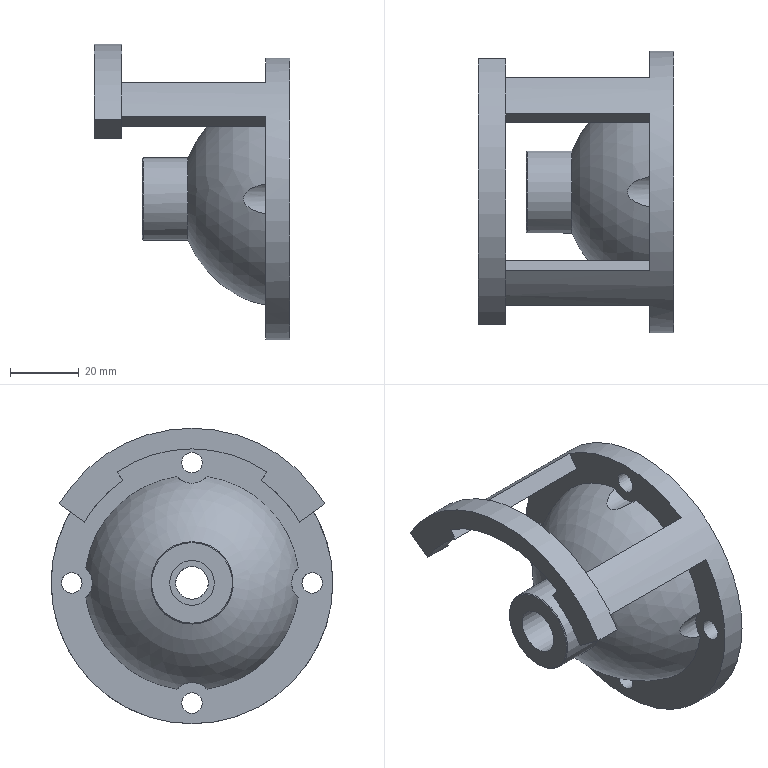Component | NX | FRONT_MOUNT_END_CAP | 1 solid | 33 faces | volume 61364 mm3 | cylinder 17 | plane 13 | sphere 2 | cone 1 | commonest cylinder face diameters 12 x4 6 x4 72 x2 82 x1 24 x1 54 x1 13 x1 9.5 x1